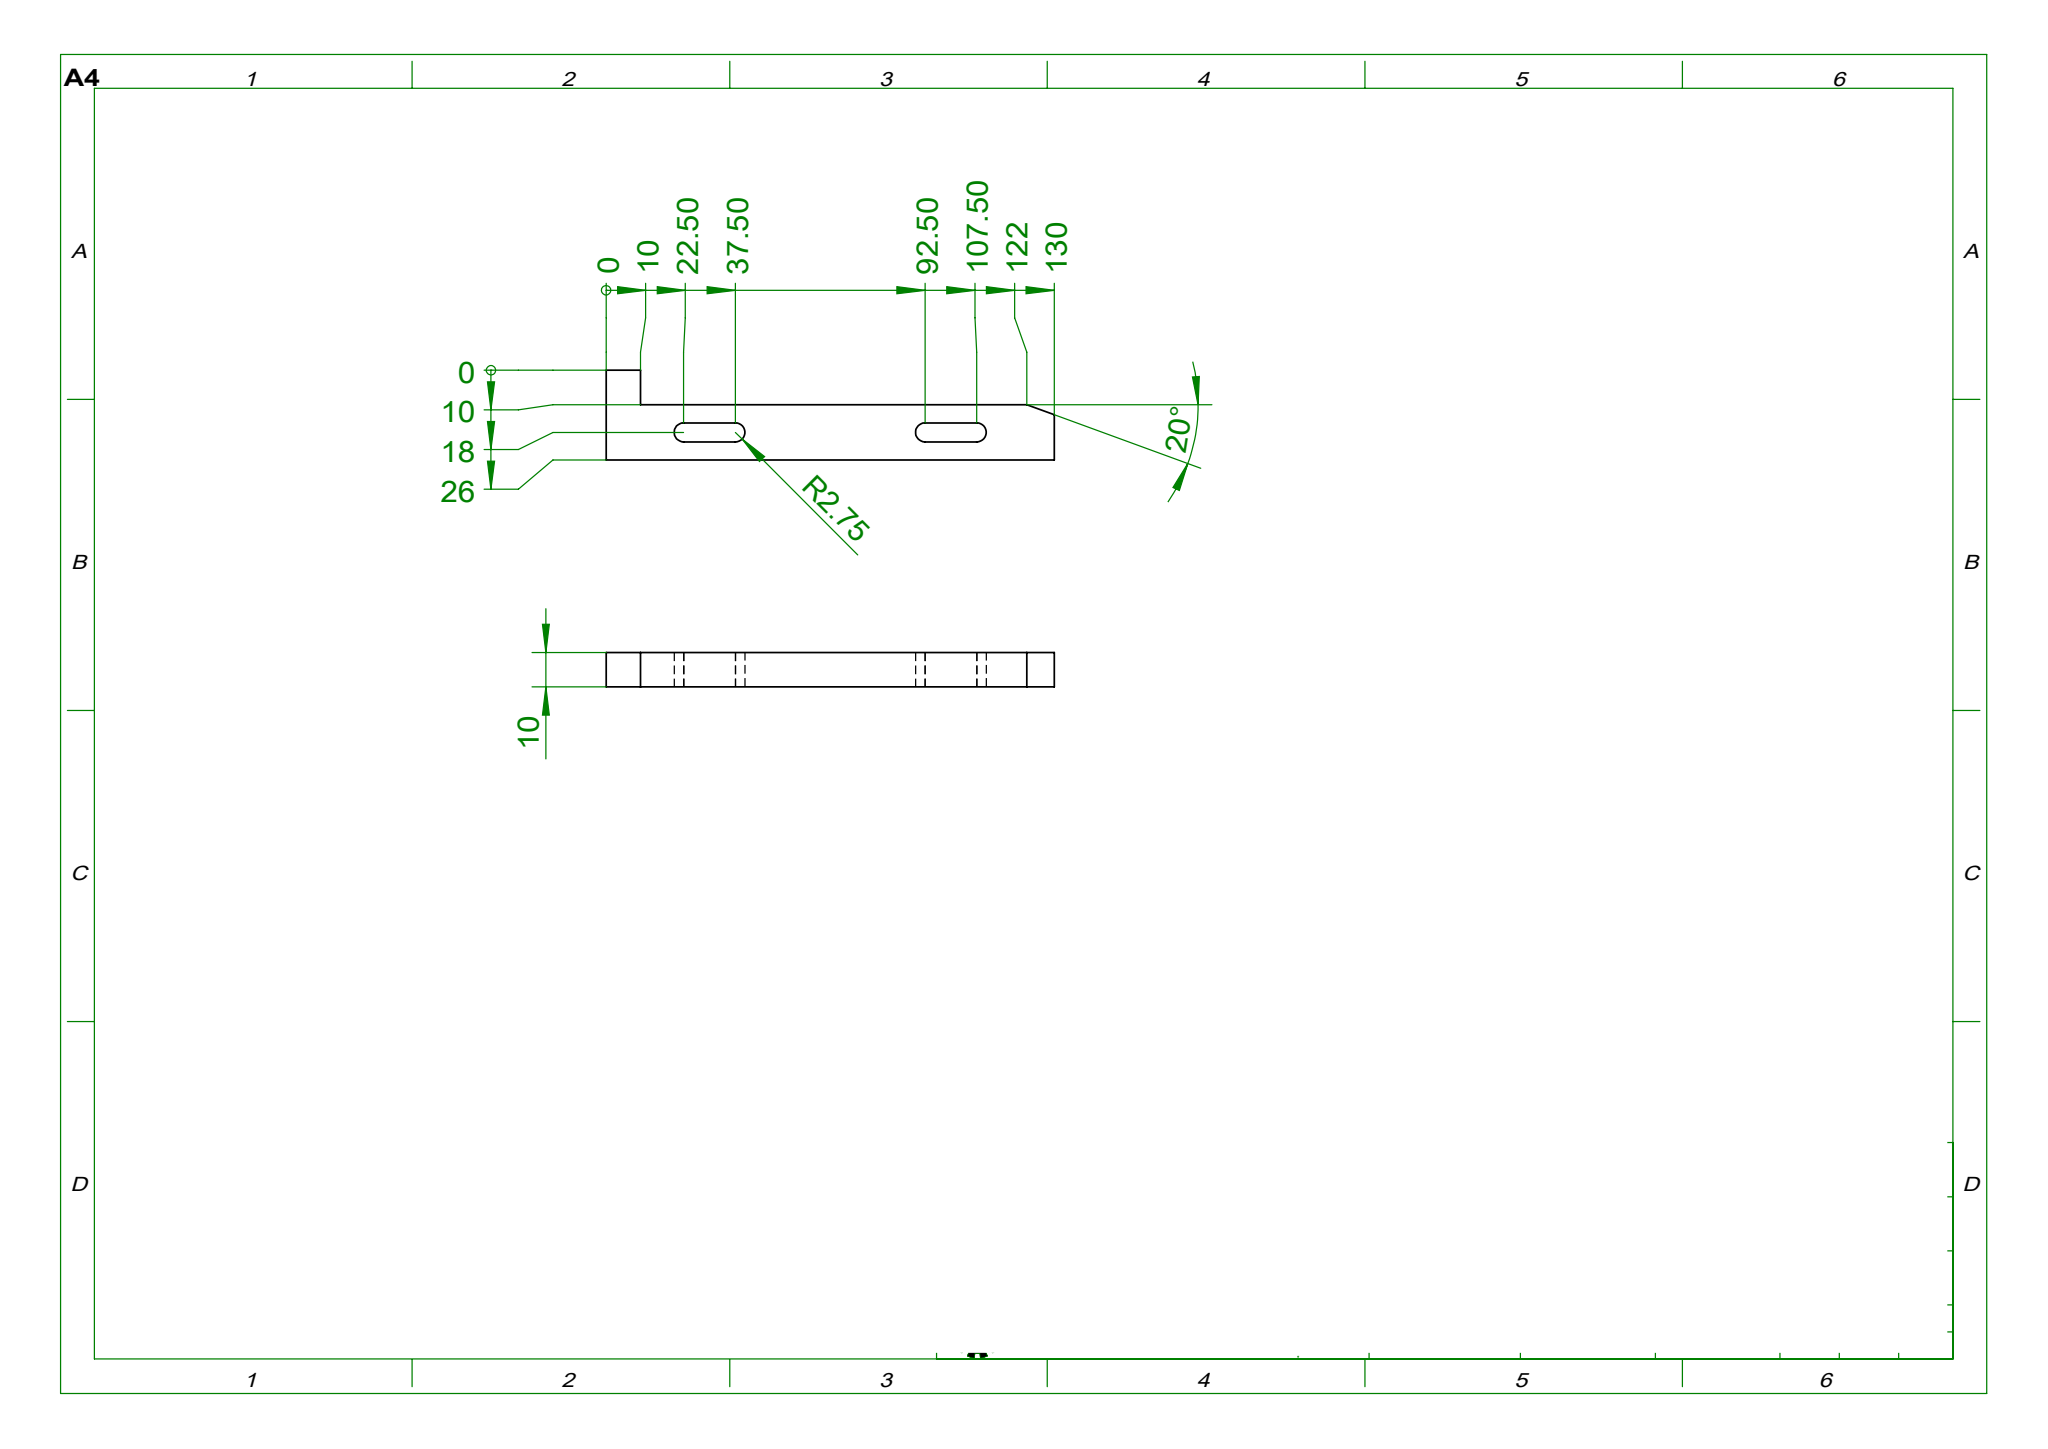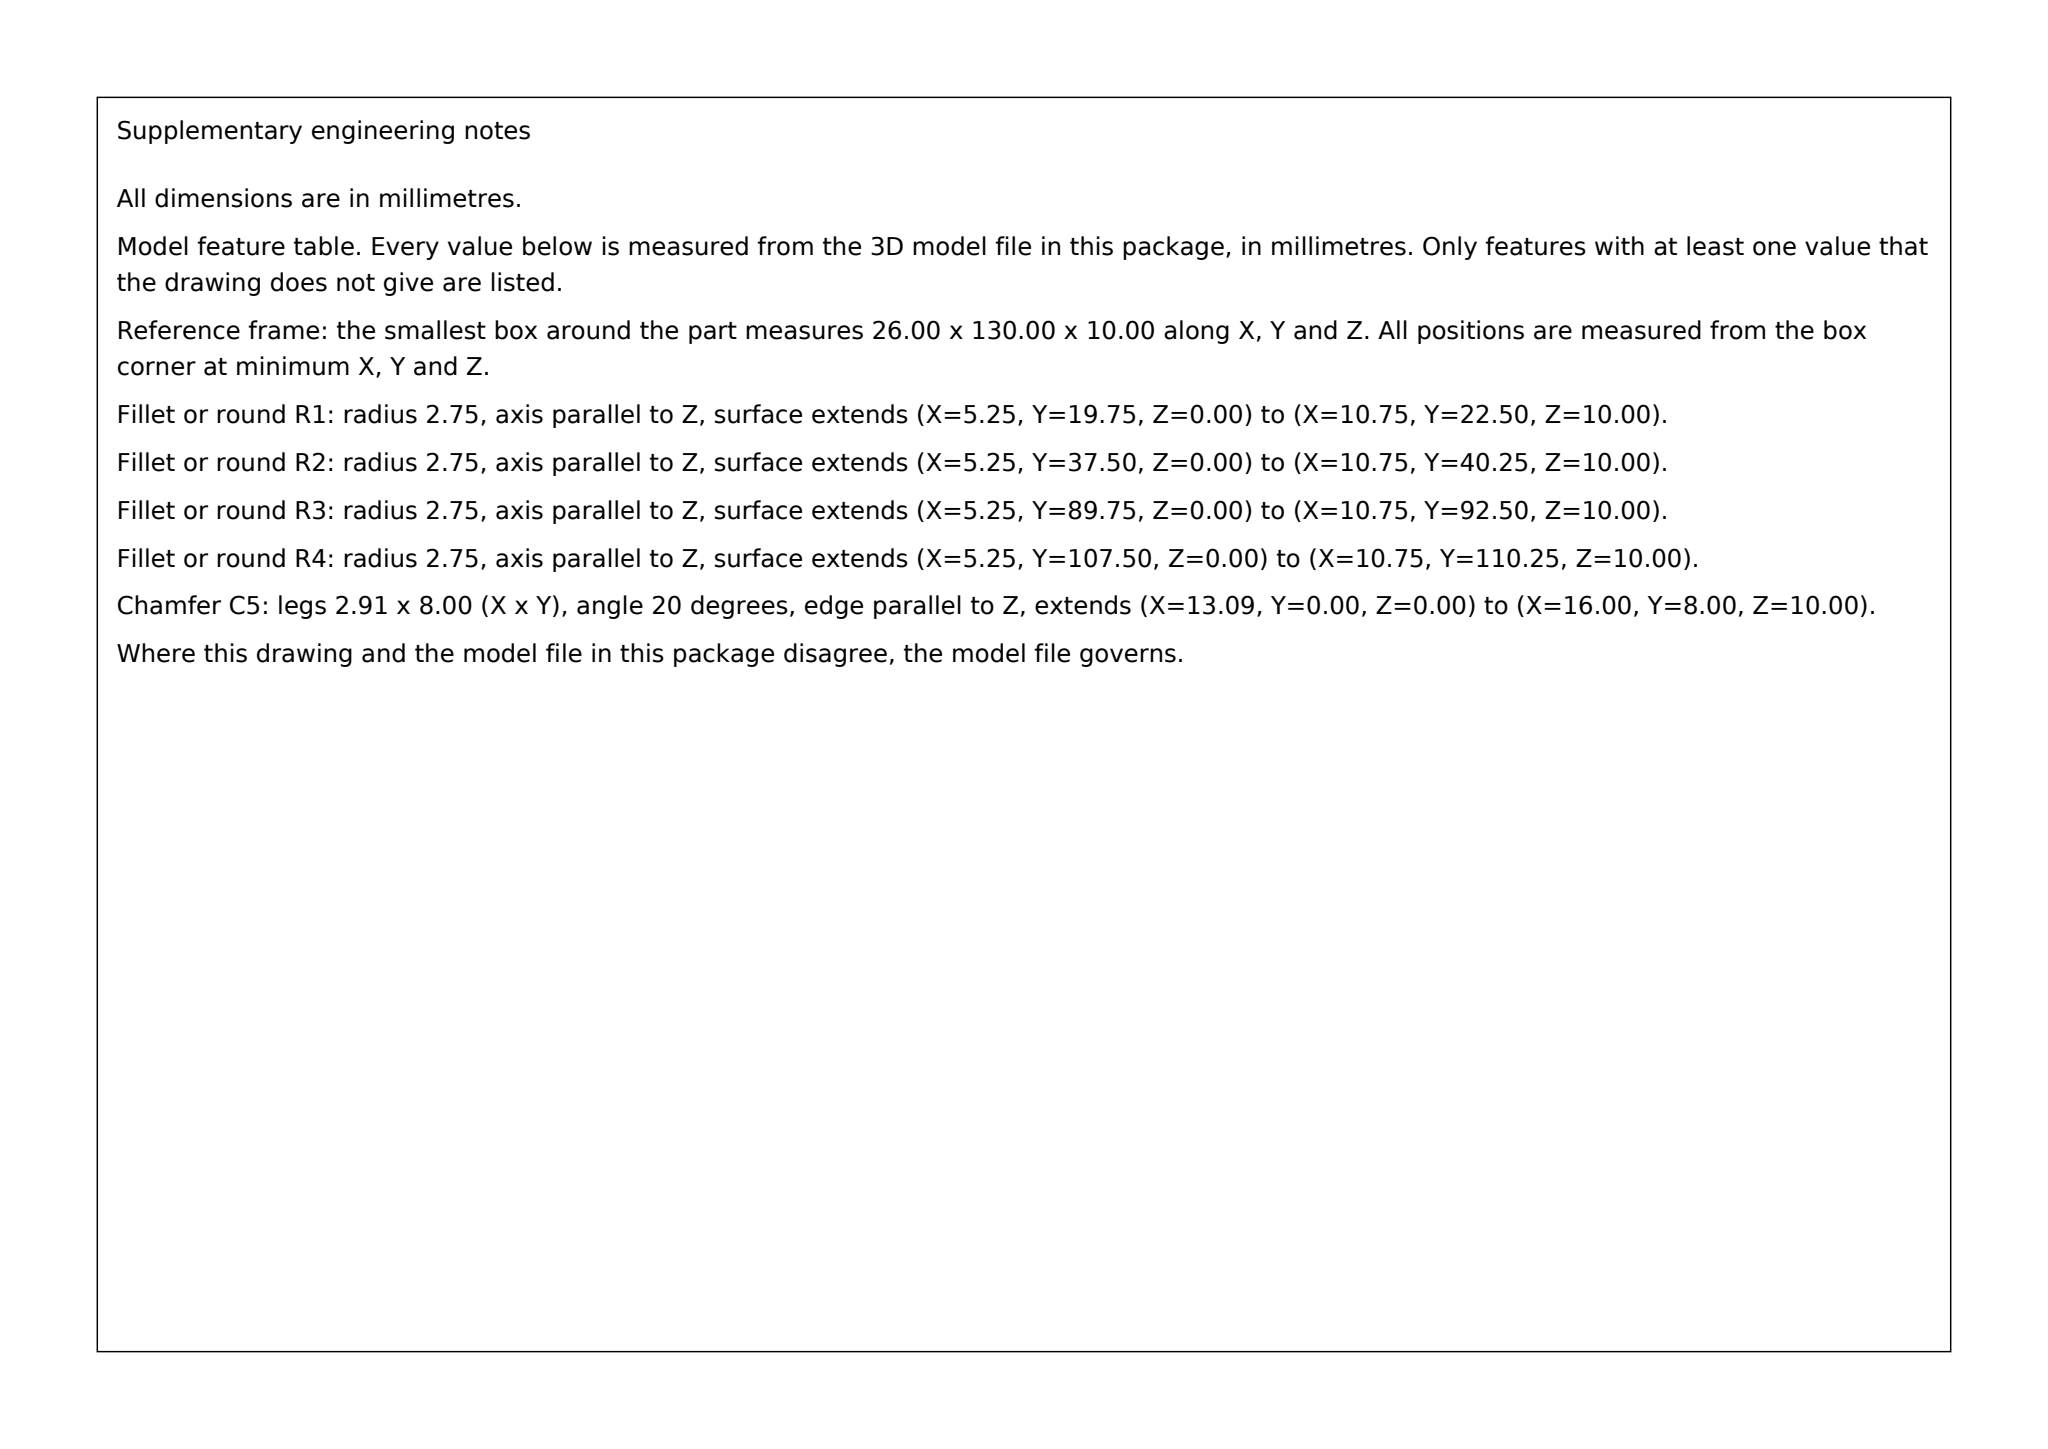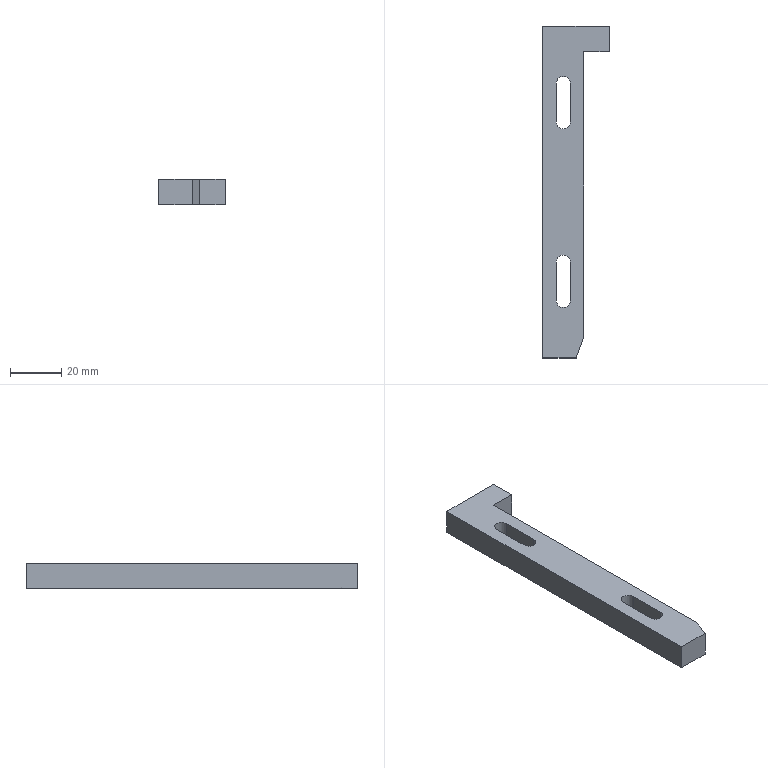Part | SolidWorks | mm | 1 solid | 17 faces | box 26 x 130 x 10 mm | volume 19558 mm3 | plane 13 | cylinder 4 | commonest cylinder face diameters 5.5 x4
build123d program:
from build123d import *

# Parameters (mm, degrees)
BOSS_EXTRUDE1_DEPTH = 10
CUT_EXTRUDE1_DEPTH  = 10
CHAMFER1_SIZE       = 8
CHAMFER1_SIZE2      = 2.912


with BuildPart() as part:
    # Sketch1 → Boss-Extrude1 (new body)
    with BuildSketch(Plane.XY):
        Polygon((16, 0), (16, 120), (26, 120), (26, 130), (0, 130), (0, 0), align=None)
    extrude(amount=BOSS_EXTRUDE1_DEPTH)

    # Sketch2 → Cut-Extrude1 (cut)
    with BuildSketch(Plane.XY.offset(10)):
        with BuildLine():
            Line((5.25, 22.5), (5.25, 37.5))
            ThreePointArc((5.25, 37.5), (8, 40.25), (10.75, 37.5))
            Line((10.75, 37.5), (10.75, 22.5))
            ThreePointArc((10.75, 22.5), (8, 19.75), (5.25, 22.5))
        make_face()
        with BuildLine():
            Line((5.25, 107.5), (5.25, 92.5))
            ThreePointArc((5.25, 92.5), (8, 89.75), (10.75, 92.5))
            Line((10.75, 92.5), (10.75, 107.5))
            ThreePointArc((10.75, 107.5), (8, 110.25), (5.25, 107.5))
        make_face()
    extrude(amount=-CUT_EXTRUDE1_DEPTH, mode=Mode.SUBTRACT)

    # Chamfer1
    chamfer1_edges = [part.edges().sort_by_distance(p)[0] for p in [
        (16, 0, 5),
    ]]
    chamfer1_side = [part.faces().sort_by_distance(p)[0] for p in [
        (16, 60, 5),
    ]]
    chamfer(chamfer1_edges, length=CHAMFER1_SIZE, length2=CHAMFER1_SIZE2, reference=chamfer1_side[0])


solid = part.part
STEP:
#1=CARTESIAN_POINT('',(0.,130.,0.));
#2=VERTEX_POINT('',#1);
#3=CARTESIAN_POINT('',(0.,0.,0.));
#4=VERTEX_POINT('',#3);
#5=CARTESIAN_POINT('',(0.,0.,0.));
#6=DIRECTION('',(0.,-1.,0.));
#7=VECTOR('',#6,1000.);
#8=LINE('',#5,#7);
#9=EDGE_CURVE('',#2,#4,#8,.T.);
#10=ORIENTED_EDGE('',*,*,#9,.T.);
#11=CARTESIAN_POINT('',(0.,0.,10.));
#12=VERTEX_POINT('',#11);
#13=CARTESIAN_POINT('',(0.,0.,10.));
#14=DIRECTION('',(0.,0.,-1.));
#15=VECTOR('',#14,1000.);
#16=LINE('',#13,#15);
#17=EDGE_CURVE('',#12,#4,#16,.T.);
#18=ORIENTED_EDGE('',*,*,#17,.F.);
#19=CARTESIAN_POINT('',(0.,130.,10.));
#20=VERTEX_POINT('',#19);
#21=CARTESIAN_POINT('',(0.,0.,10.));
#22=DIRECTION('',(0.,-1.,0.));
#23=VECTOR('',#22,1000.);
#24=LINE('',#21,#23);
#25=EDGE_CURVE('',#20,#12,#24,.T.);
#26=ORIENTED_EDGE('',*,*,#25,.F.);
#27=CARTESIAN_POINT('',(0.,130.,10.));
#28=DIRECTION('',(0.,0.,-1.));
#29=VECTOR('',#28,1000.);
#30=LINE('',#27,#29);
#31=EDGE_CURVE('',#20,#2,#30,.T.);
#32=ORIENTED_EDGE('',*,*,#31,.T.);
#33=EDGE_LOOP('',(#10,#18,#26,#32));
#34=FACE_OUTER_BOUND('',#33,.T.);
#35=CARTESIAN_POINT('',(0.,0.,10.));
#36=DIRECTION('',(1.,0.,0.));
#37=DIRECTION('',(0.,0.,-1.));
#38=AXIS2_PLACEMENT_3D('',#35,#36,#37);
#39=PLANE('',#38);
#40=ADVANCED_FACE('',(#34),#39,.F.);
#41=CARTESIAN_POINT('',(13.088,0.,0.));
#42=VERTEX_POINT('',#41);
#43=CARTESIAN_POINT('',(0.,0.,0.));
#44=DIRECTION('',(1.,0.,0.));
#45=VECTOR('',#44,1000.);
#46=LINE('',#43,#45);
#47=EDGE_CURVE('',#4,#42,#46,.T.);
#48=ORIENTED_EDGE('',*,*,#47,.T.);
#49=CARTESIAN_POINT('',(13.088,-0.,10.));
#50=VERTEX_POINT('',#49);
#51=CARTESIAN_POINT('',(13.088,0.,10.));
#52=DIRECTION('',(0.,0.,1.));
#53=VECTOR('',#52,1000.);
#54=LINE('',#51,#53);
#55=EDGE_CURVE('',#42,#50,#54,.T.);
#56=ORIENTED_EDGE('',*,*,#55,.T.);
#57=CARTESIAN_POINT('',(0.,0.,10.));
#58=DIRECTION('',(1.,0.,0.));
#59=VECTOR('',#58,1000.);
#60=LINE('',#57,#59);
#61=EDGE_CURVE('',#12,#50,#60,.T.);
#62=ORIENTED_EDGE('',*,*,#61,.F.);
#63=ORIENTED_EDGE('',*,*,#17,.T.);
#64=EDGE_LOOP('',(#48,#56,#62,#63));
#65=FACE_OUTER_BOUND('',#64,.T.);
#66=CARTESIAN_POINT('',(0.,0.,10.));
#67=DIRECTION('',(0.,1.,0.));
#68=DIRECTION('',(0.,0.,1.));
#69=AXIS2_PLACEMENT_3D('',#66,#67,#68);
#70=PLANE('',#69);
#71=ADVANCED_FACE('',(#65),#70,.F.);
#72=CARTESIAN_POINT('',(16.,8.,10.));
#73=VERTEX_POINT('',#72);
#74=CARTESIAN_POINT('',(16.,120.,10.));
#75=VERTEX_POINT('',#74);
#76=CARTESIAN_POINT('',(16.,0.,10.));
#77=DIRECTION('',(0.,1.,0.));
#78=VECTOR('',#77,1000.);
#79=LINE('',#76,#78);
#80=EDGE_CURVE('',#73,#75,#79,.T.);
#81=ORIENTED_EDGE('',*,*,#80,.F.);
#82=CARTESIAN_POINT('',(16.,8.,0.));
#83=VERTEX_POINT('',#82);
#84=CARTESIAN_POINT('',(16.,8.,10.));
#85=DIRECTION('',(0.,0.,-1.));
#86=VECTOR('',#85,1000.);
#87=LINE('',#84,#86);
#88=EDGE_CURVE('',#73,#83,#87,.T.);
#89=ORIENTED_EDGE('',*,*,#88,.T.);
#90=CARTESIAN_POINT('',(16.,120.,0.));
#91=VERTEX_POINT('',#90);
#92=CARTESIAN_POINT('',(16.,0.,0.));
#93=DIRECTION('',(0.,1.,0.));
#94=VECTOR('',#93,1000.);
#95=LINE('',#92,#94);
#96=EDGE_CURVE('',#83,#91,#95,.T.);
#97=ORIENTED_EDGE('',*,*,#96,.T.);
#98=CARTESIAN_POINT('',(16.,120.,10.));
#99=DIRECTION('',(0.,0.,-1.));
#100=VECTOR('',#99,1000.);
#101=LINE('',#98,#100);
#102=EDGE_CURVE('',#75,#91,#101,.T.);
#103=ORIENTED_EDGE('',*,*,#102,.F.);
#104=EDGE_LOOP('',(#81,#89,#97,#103));
#105=FACE_OUTER_BOUND('',#104,.T.);
#106=CARTESIAN_POINT('',(16.,0.,10.));
#107=DIRECTION('',(-1.,0.,0.));
#108=DIRECTION('',(0.,0.,1.));
#109=AXIS2_PLACEMENT_3D('',#106,#107,#108);
#110=PLANE('',#109);
#111=ADVANCED_FACE('',(#105),#110,.F.);
#112=CARTESIAN_POINT('',(26.,120.,0.));
#113=VERTEX_POINT('',#112);
#114=CARTESIAN_POINT('',(16.,120.,0.));
#115=DIRECTION('',(1.,0.,0.));
#116=VECTOR('',#115,1000.);
#117=LINE('',#114,#116);
#118=EDGE_CURVE('',#91,#113,#117,.T.);
#119=ORIENTED_EDGE('',*,*,#118,.T.);
#120=CARTESIAN_POINT('',(26.,120.,10.));
#121=VERTEX_POINT('',#120);
#122=CARTESIAN_POINT('',(26.,120.,10.));
#123=DIRECTION('',(0.,0.,-1.));
#124=VECTOR('',#123,1000.);
#125=LINE('',#122,#124);
#126=EDGE_CURVE('',#121,#113,#125,.T.);
#127=ORIENTED_EDGE('',*,*,#126,.F.);
#128=CARTESIAN_POINT('',(16.,120.,10.));
#129=DIRECTION('',(1.,0.,0.));
#130=VECTOR('',#129,1000.);
#131=LINE('',#128,#130);
#132=EDGE_CURVE('',#75,#121,#131,.T.);
#133=ORIENTED_EDGE('',*,*,#132,.F.);
#134=ORIENTED_EDGE('',*,*,#102,.T.);
#135=EDGE_LOOP('',(#119,#127,#133,#134));
#136=FACE_OUTER_BOUND('',#135,.T.);
#137=CARTESIAN_POINT('',(16.,120.,10.));
#138=DIRECTION('',(0.,1.,0.));
#139=DIRECTION('',(0.,0.,1.));
#140=AXIS2_PLACEMENT_3D('',#137,#138,#139);
#141=PLANE('',#140);
#142=ADVANCED_FACE('',(#136),#141,.F.);
#143=CARTESIAN_POINT('',(26.,130.,0.));
#144=VERTEX_POINT('',#143);
#145=CARTESIAN_POINT('',(26.,120.,0.));
#146=DIRECTION('',(0.,1.,0.));
#147=VECTOR('',#146,1000.);
#148=LINE('',#145,#147);
#149=EDGE_CURVE('',#113,#144,#148,.T.);
#150=ORIENTED_EDGE('',*,*,#149,.T.);
#151=CARTESIAN_POINT('',(26.,130.,10.));
#152=VERTEX_POINT('',#151);
#153=CARTESIAN_POINT('',(26.,130.,10.));
#154=DIRECTION('',(0.,0.,-1.));
#155=VECTOR('',#154,1000.);
#156=LINE('',#153,#155);
#157=EDGE_CURVE('',#152,#144,#156,.T.);
#158=ORIENTED_EDGE('',*,*,#157,.F.);
#159=CARTESIAN_POINT('',(26.,120.,10.));
#160=DIRECTION('',(0.,1.,0.));
#161=VECTOR('',#160,1000.);
#162=LINE('',#159,#161);
#163=EDGE_CURVE('',#121,#152,#162,.T.);
#164=ORIENTED_EDGE('',*,*,#163,.F.);
#165=ORIENTED_EDGE('',*,*,#126,.T.);
#166=EDGE_LOOP('',(#150,#158,#164,#165));
#167=FACE_OUTER_BOUND('',#166,.T.);
#168=CARTESIAN_POINT('',(26.,120.,10.));
#169=DIRECTION('',(-1.,0.,0.));
#170=DIRECTION('',(0.,0.,1.));
#171=AXIS2_PLACEMENT_3D('',#168,#169,#170);
#172=PLANE('',#171);
#173=ADVANCED_FACE('',(#167),#172,.F.);
#174=CARTESIAN_POINT('',(0.,130.,0.));
#175=DIRECTION('',(-1.,0.,0.));
#176=VECTOR('',#175,1000.);
#177=LINE('',#174,#176);
#178=EDGE_CURVE('',#144,#2,#177,.T.);
#179=ORIENTED_EDGE('',*,*,#178,.T.);
#180=ORIENTED_EDGE('',*,*,#31,.F.);
#181=CARTESIAN_POINT('',(0.,130.,10.));
#182=DIRECTION('',(-1.,0.,0.));
#183=VECTOR('',#182,1000.);
#184=LINE('',#181,#183);
#185=EDGE_CURVE('',#152,#20,#184,.T.);
#186=ORIENTED_EDGE('',*,*,#185,.F.);
#187=ORIENTED_EDGE('',*,*,#157,.T.);
#188=EDGE_LOOP('',(#179,#180,#186,#187));
#189=FACE_OUTER_BOUND('',#188,.T.);
#190=CARTESIAN_POINT('',(0.,130.,10.));
#191=DIRECTION('',(0.,-1.,0.));
#192=DIRECTION('',(0.,0.,-1.));
#193=AXIS2_PLACEMENT_3D('',#190,#191,#192);
#194=PLANE('',#193);
#195=ADVANCED_FACE('',(#189),#194,.F.);
#196=CARTESIAN_POINT('',(5.25,107.5,10.));
#197=VERTEX_POINT('',#196);
#198=CARTESIAN_POINT('',(5.25,92.5,10.));
#199=VERTEX_POINT('',#198);
#200=CARTESIAN_POINT('',(5.25,107.5,10.));
#201=DIRECTION('',(0.,-1.,0.));
#202=VECTOR('',#201,1000.);
#203=LINE('',#200,#202);
#204=EDGE_CURVE('',#197,#199,#203,.T.);
#205=ORIENTED_EDGE('',*,*,#204,.F.);
#206=CARTESIAN_POINT('',(10.75,107.5,10.));
#207=VERTEX_POINT('',#206);
#208=CARTESIAN_POINT('',(8.,107.5,10.));
#209=DIRECTION('',(0.,0.,1.));
#210=DIRECTION('',(-1.,0.,0.));
#211=AXIS2_PLACEMENT_3D('',#208,#209,#210);
#212=CIRCLE('',#211,2.75);
#213=EDGE_CURVE('',#207,#197,#212,.T.);
#214=ORIENTED_EDGE('',*,*,#213,.F.);
#215=CARTESIAN_POINT('',(10.75,92.5,10.));
#216=VERTEX_POINT('',#215);
#217=CARTESIAN_POINT('',(10.75,107.5,10.));
#218=DIRECTION('',(-0.,1.,0.));
#219=VECTOR('',#218,1000.);
#220=LINE('',#217,#219);
#221=EDGE_CURVE('',#216,#207,#220,.T.);
#222=ORIENTED_EDGE('',*,*,#221,.F.);
#223=CARTESIAN_POINT('',(8.,92.5,10.));
#224=DIRECTION('',(0.,0.,1.));
#225=DIRECTION('',(-1.,0.,0.));
#226=AXIS2_PLACEMENT_3D('',#223,#224,#225);
#227=CIRCLE('',#226,2.75);
#228=EDGE_CURVE('',#199,#216,#227,.T.);
#229=ORIENTED_EDGE('',*,*,#228,.F.);
#230=EDGE_LOOP('',(#205,#214,#222,#229));
#231=FACE_BOUND('',#230,.T.);
#232=CARTESIAN_POINT('',(10.75,22.5,10.));
#233=VERTEX_POINT('',#232);
#234=CARTESIAN_POINT('',(10.75,37.5,10.));
#235=VERTEX_POINT('',#234);
#236=CARTESIAN_POINT('',(10.75,22.5,10.));
#237=DIRECTION('',(0.,1.,0.));
#238=VECTOR('',#237,1000.);
#239=LINE('',#236,#238);
#240=EDGE_CURVE('',#233,#235,#239,.T.);
#241=ORIENTED_EDGE('',*,*,#240,.F.);
#242=CARTESIAN_POINT('',(5.25,22.5,10.));
#243=VERTEX_POINT('',#242);
#244=CARTESIAN_POINT('',(8.,22.5,10.));
#245=DIRECTION('',(0.,0.,1.));
#246=DIRECTION('',(1.,0.,0.));
#247=AXIS2_PLACEMENT_3D('',#244,#245,#246);
#248=CIRCLE('',#247,2.75);
#249=EDGE_CURVE('',#243,#233,#248,.T.);
#250=ORIENTED_EDGE('',*,*,#249,.F.);
#251=CARTESIAN_POINT('',(5.25,37.5,10.));
#252=VERTEX_POINT('',#251);
#253=CARTESIAN_POINT('',(5.25,22.5,10.));
#254=DIRECTION('',(-0.,-1.,0.));
#255=VECTOR('',#254,1000.);
#256=LINE('',#253,#255);
#257=EDGE_CURVE('',#252,#243,#256,.T.);
#258=ORIENTED_EDGE('',*,*,#257,.F.);
#259=CARTESIAN_POINT('',(8.,37.5,10.));
#260=DIRECTION('',(0.,0.,1.));
#261=DIRECTION('',(1.,0.,0.));
#262=AXIS2_PLACEMENT_3D('',#259,#260,#261);
#263=CIRCLE('',#262,2.75);
#264=EDGE_CURVE('',#235,#252,#263,.T.);
#265=ORIENTED_EDGE('',*,*,#264,.F.);
#266=EDGE_LOOP('',(#241,#250,#258,#265));
#267=FACE_BOUND('',#266,.T.);
#268=ORIENTED_EDGE('',*,*,#61,.T.);
#269=CARTESIAN_POINT('',(16.,8.,10.));
#270=DIRECTION('',(0.342,0.9397,0.));
#271=VECTOR('',#270,1000.);
#272=LINE('',#269,#271);
#273=EDGE_CURVE('',#50,#73,#272,.T.);
#274=ORIENTED_EDGE('',*,*,#273,.T.);
#275=ORIENTED_EDGE('',*,*,#80,.T.);
#276=ORIENTED_EDGE('',*,*,#132,.T.);
#277=ORIENTED_EDGE('',*,*,#163,.T.);
#278=ORIENTED_EDGE('',*,*,#185,.T.);
#279=ORIENTED_EDGE('',*,*,#25,.T.);
#280=EDGE_LOOP('',(#268,#274,#275,#276,#277,#278,#279));
#281=FACE_OUTER_BOUND('',#280,.T.);
#282=CARTESIAN_POINT('',(0.,0.,10.));
#283=DIRECTION('',(0.,0.,-1.));
#284=DIRECTION('',(-1.,0.,0.));
#285=AXIS2_PLACEMENT_3D('',#282,#283,#284);
#286=PLANE('',#285);
#287=ADVANCED_FACE('',(#231,#267,#281),#286,.F.);
#288=CARTESIAN_POINT('',(10.75,107.5,0.));
#289=VERTEX_POINT('',#288);
#290=CARTESIAN_POINT('',(5.25,107.5,0.));
#291=VERTEX_POINT('',#290);
#292=CARTESIAN_POINT('',(8.,107.5,0.));
#293=DIRECTION('',(0.,0.,1.));
#294=DIRECTION('',(-1.,0.,0.));
#295=AXIS2_PLACEMENT_3D('',#292,#293,#294);
#296=CIRCLE('',#295,2.75);
#297=EDGE_CURVE('',#289,#291,#296,.T.);
#298=ORIENTED_EDGE('',*,*,#297,.T.);
#299=CARTESIAN_POINT('',(5.25,92.5,0.));
#300=VERTEX_POINT('',#299);
#301=CARTESIAN_POINT('',(5.25,107.5,0.));
#302=DIRECTION('',(0.,-1.,0.));
#303=VECTOR('',#302,1000.);
#304=LINE('',#301,#303);
#305=EDGE_CURVE('',#291,#300,#304,.T.);
#306=ORIENTED_EDGE('',*,*,#305,.T.);
#307=CARTESIAN_POINT('',(10.75,92.5,0.));
#308=VERTEX_POINT('',#307);
#309=CARTESIAN_POINT('',(8.,92.5,0.));
#310=DIRECTION('',(0.,0.,1.));
#311=DIRECTION('',(-1.,0.,0.));
#312=AXIS2_PLACEMENT_3D('',#309,#310,#311);
#313=CIRCLE('',#312,2.75);
#314=EDGE_CURVE('',#300,#308,#313,.T.);
#315=ORIENTED_EDGE('',*,*,#314,.T.);
#316=CARTESIAN_POINT('',(10.75,107.5,0.));
#317=DIRECTION('',(-0.,1.,0.));
#318=VECTOR('',#317,1000.);
#319=LINE('',#316,#318);
#320=EDGE_CURVE('',#308,#289,#319,.T.);
#321=ORIENTED_EDGE('',*,*,#320,.T.);
#322=EDGE_LOOP('',(#298,#306,#315,#321));
#323=FACE_BOUND('',#322,.T.);
#324=CARTESIAN_POINT('',(5.25,22.5,0.));
#325=VERTEX_POINT('',#324);
#326=CARTESIAN_POINT('',(10.75,22.5,0.));
#327=VERTEX_POINT('',#326);
#328=CARTESIAN_POINT('',(8.,22.5,0.));
#329=DIRECTION('',(0.,0.,1.));
#330=DIRECTION('',(1.,0.,0.));
#331=AXIS2_PLACEMENT_3D('',#328,#329,#330);
#332=CIRCLE('',#331,2.75);
#333=EDGE_CURVE('',#325,#327,#332,.T.);
#334=ORIENTED_EDGE('',*,*,#333,.T.);
#335=CARTESIAN_POINT('',(10.75,37.5,0.));
#336=VERTEX_POINT('',#335);
#337=CARTESIAN_POINT('',(10.75,22.5,0.));
#338=DIRECTION('',(0.,1.,0.));
#339=VECTOR('',#338,1000.);
#340=LINE('',#337,#339);
#341=EDGE_CURVE('',#327,#336,#340,.T.);
#342=ORIENTED_EDGE('',*,*,#341,.T.);
#343=CARTESIAN_POINT('',(5.25,37.5,0.));
#344=VERTEX_POINT('',#343);
#345=CARTESIAN_POINT('',(8.,37.5,0.));
#346=DIRECTION('',(0.,0.,1.));
#347=DIRECTION('',(1.,0.,0.));
#348=AXIS2_PLACEMENT_3D('',#345,#346,#347);
#349=CIRCLE('',#348,2.75);
#350=EDGE_CURVE('',#336,#344,#349,.T.);
#351=ORIENTED_EDGE('',*,*,#350,.T.);
#352=CARTESIAN_POINT('',(5.25,22.5,0.));
#353=DIRECTION('',(-0.,-1.,0.));
#354=VECTOR('',#353,1000.);
#355=LINE('',#352,#354);
#356=EDGE_CURVE('',#344,#325,#355,.T.);
#357=ORIENTED_EDGE('',*,*,#356,.T.);
#358=EDGE_LOOP('',(#334,#342,#351,#357));
#359=FACE_BOUND('',#358,.T.);
#360=ORIENTED_EDGE('',*,*,#96,.F.);
#361=CARTESIAN_POINT('',(11.557,-4.206,0.));
#362=DIRECTION('',(-0.342,-0.9397,0.));
#363=VECTOR('',#362,1000.);
#364=LINE('',#361,#363);
#365=EDGE_CURVE('',#83,#42,#364,.T.);
#366=ORIENTED_EDGE('',*,*,#365,.T.);
#367=ORIENTED_EDGE('',*,*,#47,.F.);
#368=ORIENTED_EDGE('',*,*,#9,.F.);
#369=ORIENTED_EDGE('',*,*,#178,.F.);
#370=ORIENTED_EDGE('',*,*,#149,.F.);
#371=ORIENTED_EDGE('',*,*,#118,.F.);
#372=EDGE_LOOP('',(#360,#366,#367,#368,#369,#370,#371));
#373=FACE_OUTER_BOUND('',#372,.T.);
#374=CARTESIAN_POINT('',(0.,0.,0.));
#375=DIRECTION('',(0.,0.,-1.));
#376=DIRECTION('',(-1.,0.,0.));
#377=AXIS2_PLACEMENT_3D('',#374,#375,#376);
#378=PLANE('',#377);
#379=ADVANCED_FACE('',(#323,#359,#373),#378,.T.);
#380=ORIENTED_EDGE('',*,*,#249,.T.);
#381=CARTESIAN_POINT('',(10.75,22.5,0.));
#382=DIRECTION('',(0.,0.,1.));
#383=VECTOR('',#382,1000.);
#384=LINE('',#381,#383);
#385=EDGE_CURVE('',#327,#233,#384,.T.);
#386=ORIENTED_EDGE('',*,*,#385,.F.);
#387=ORIENTED_EDGE('',*,*,#333,.F.);
#388=CARTESIAN_POINT('',(5.25,22.5,0.));
#389=DIRECTION('',(0.,0.,1.));
#390=VECTOR('',#389,1000.);
#391=LINE('',#388,#390);
#392=EDGE_CURVE('',#325,#243,#391,.T.);
#393=ORIENTED_EDGE('',*,*,#392,.T.);
#394=EDGE_LOOP('',(#380,#386,#387,#393));
#395=FACE_OUTER_BOUND('',#394,.T.);
#396=CARTESIAN_POINT('',(8.,22.5,0.));
#397=DIRECTION('',(0.,0.,1.));
#398=DIRECTION('',(1.,0.,0.));
#399=AXIS2_PLACEMENT_3D('',#396,#397,#398);
#400=CYLINDRICAL_SURFACE('',#399,2.75);
#401=ADVANCED_FACE('',(#395),#400,.F.);
#402=ORIENTED_EDGE('',*,*,#257,.T.);
#403=ORIENTED_EDGE('',*,*,#392,.F.);
#404=ORIENTED_EDGE('',*,*,#356,.F.);
#405=CARTESIAN_POINT('',(5.25,37.5,0.));
#406=DIRECTION('',(0.,0.,1.));
#407=VECTOR('',#406,1000.);
#408=LINE('',#405,#407);
#409=EDGE_CURVE('',#344,#252,#408,.T.);
#410=ORIENTED_EDGE('',*,*,#409,.T.);
#411=EDGE_LOOP('',(#402,#403,#404,#410));
#412=FACE_OUTER_BOUND('',#411,.T.);
#413=CARTESIAN_POINT('',(5.25,22.5,0.));
#414=DIRECTION('',(-1.,0.,0.));
#415=DIRECTION('',(-0.,-1.,0.));
#416=AXIS2_PLACEMENT_3D('',#413,#414,#415);
#417=PLANE('',#416);
#418=ADVANCED_FACE('',(#412),#417,.F.);
#419=ORIENTED_EDGE('',*,*,#264,.T.);
#420=ORIENTED_EDGE('',*,*,#409,.F.);
#421=ORIENTED_EDGE('',*,*,#350,.F.);
#422=CARTESIAN_POINT('',(10.75,37.5,0.));
#423=DIRECTION('',(0.,0.,1.));
#424=VECTOR('',#423,1000.);
#425=LINE('',#422,#424);
#426=EDGE_CURVE('',#336,#235,#425,.T.);
#427=ORIENTED_EDGE('',*,*,#426,.T.);
#428=EDGE_LOOP('',(#419,#420,#421,#427));
#429=FACE_OUTER_BOUND('',#428,.T.);
#430=CARTESIAN_POINT('',(8.,37.5,0.));
#431=DIRECTION('',(0.,0.,1.));
#432=DIRECTION('',(1.,0.,0.));
#433=AXIS2_PLACEMENT_3D('',#430,#431,#432);
#434=CYLINDRICAL_SURFACE('',#433,2.75);
#435=ADVANCED_FACE('',(#429),#434,.F.);
#436=ORIENTED_EDGE('',*,*,#240,.T.);
#437=ORIENTED_EDGE('',*,*,#426,.F.);
#438=ORIENTED_EDGE('',*,*,#341,.F.);
#439=ORIENTED_EDGE('',*,*,#385,.T.);
#440=EDGE_LOOP('',(#436,#437,#438,#439));
#441=FACE_OUTER_BOUND('',#440,.T.);
#442=CARTESIAN_POINT('',(10.75,22.5,0.));
#443=DIRECTION('',(1.,-0.,0.));
#444=DIRECTION('',(0.,1.,0.));
#445=AXIS2_PLACEMENT_3D('',#442,#443,#444);
#446=PLANE('',#445);
#447=ADVANCED_FACE('',(#441),#446,.F.);
#448=ORIENTED_EDGE('',*,*,#213,.T.);
#449=CARTESIAN_POINT('',(5.25,107.5,0.));
#450=DIRECTION('',(0.,0.,1.));
#451=VECTOR('',#450,1000.);
#452=LINE('',#449,#451);
#453=EDGE_CURVE('',#291,#197,#452,.T.);
#454=ORIENTED_EDGE('',*,*,#453,.F.);
#455=ORIENTED_EDGE('',*,*,#297,.F.);
#456=CARTESIAN_POINT('',(10.75,107.5,0.));
#457=DIRECTION('',(0.,0.,1.));
#458=VECTOR('',#457,1000.);
#459=LINE('',#456,#458);
#460=EDGE_CURVE('',#289,#207,#459,.T.);
#461=ORIENTED_EDGE('',*,*,#460,.T.);
#462=EDGE_LOOP('',(#448,#454,#455,#461));
#463=FACE_OUTER_BOUND('',#462,.T.);
#464=CARTESIAN_POINT('',(8.,107.5,0.));
#465=DIRECTION('',(0.,0.,1.));
#466=DIRECTION('',(1.,0.,0.));
#467=AXIS2_PLACEMENT_3D('',#464,#465,#466);
#468=CYLINDRICAL_SURFACE('',#467,2.75);
#469=ADVANCED_FACE('',(#463),#468,.F.);
#470=ORIENTED_EDGE('',*,*,#221,.T.);
#471=ORIENTED_EDGE('',*,*,#460,.F.);
#472=ORIENTED_EDGE('',*,*,#320,.F.);
#473=CARTESIAN_POINT('',(10.75,92.5,0.));
#474=DIRECTION('',(0.,0.,1.));
#475=VECTOR('',#474,1000.);
#476=LINE('',#473,#475);
#477=EDGE_CURVE('',#308,#216,#476,.T.);
#478=ORIENTED_EDGE('',*,*,#477,.T.);
#479=EDGE_LOOP('',(#470,#471,#472,#478));
#480=FACE_OUTER_BOUND('',#479,.T.);
#481=CARTESIAN_POINT('',(10.75,107.5,0.));
#482=DIRECTION('',(1.,0.,0.));
#483=DIRECTION('',(-0.,1.,0.));
#484=AXIS2_PLACEMENT_3D('',#481,#482,#483);
#485=PLANE('',#484);
#486=ADVANCED_FACE('',(#480),#485,.F.);
#487=ORIENTED_EDGE('',*,*,#228,.T.);
#488=ORIENTED_EDGE('',*,*,#477,.F.);
#489=ORIENTED_EDGE('',*,*,#314,.F.);
#490=CARTESIAN_POINT('',(5.25,92.5,0.));
#491=DIRECTION('',(0.,0.,1.));
#492=VECTOR('',#491,1000.);
#493=LINE('',#490,#492);
#494=EDGE_CURVE('',#300,#199,#493,.T.);
#495=ORIENTED_EDGE('',*,*,#494,.T.);
#496=EDGE_LOOP('',(#487,#488,#489,#495));
#497=FACE_OUTER_BOUND('',#496,.T.);
#498=CARTESIAN_POINT('',(8.,92.5,0.));
#499=DIRECTION('',(0.,0.,1.));
#500=DIRECTION('',(1.,0.,0.));
#501=AXIS2_PLACEMENT_3D('',#498,#499,#500);
#502=CYLINDRICAL_SURFACE('',#501,2.75);
#503=ADVANCED_FACE('',(#497),#502,.F.);
#504=ORIENTED_EDGE('',*,*,#204,.T.);
#505=ORIENTED_EDGE('',*,*,#494,.F.);
#506=ORIENTED_EDGE('',*,*,#305,.F.);
#507=ORIENTED_EDGE('',*,*,#453,.T.);
#508=EDGE_LOOP('',(#504,#505,#506,#507));
#509=FACE_OUTER_BOUND('',#508,.T.);
#510=CARTESIAN_POINT('',(5.25,107.5,0.));
#511=DIRECTION('',(-1.,-0.,0.));
#512=DIRECTION('',(0.,-1.,0.));
#513=AXIS2_PLACEMENT_3D('',#510,#511,#512);
#514=PLANE('',#513);
#515=ADVANCED_FACE('',(#509),#514,.F.);
#516=ORIENTED_EDGE('',*,*,#273,.F.);
#517=ORIENTED_EDGE('',*,*,#55,.F.);
#518=ORIENTED_EDGE('',*,*,#365,.F.);
#519=ORIENTED_EDGE('',*,*,#88,.F.);
#520=EDGE_LOOP('',(#516,#517,#518,#519));
#521=FACE_OUTER_BOUND('',#520,.T.);
#522=CARTESIAN_POINT('',(16.,8.,10.));
#523=DIRECTION('',(-0.9397,0.342,0.));
#524=DIRECTION('',(0.,0.,-1.));
#525=AXIS2_PLACEMENT_3D('',#522,#523,#524);
#526=PLANE('',#525);
#527=ADVANCED_FACE('',(#521),#526,.F.);
#528=CLOSED_SHELL('',(#40,#71,#111,#142,#173,#195,#287,#379,#401,#418,#435,#447,#469,#486,#503,#515,#527));
#529=MANIFOLD_SOLID_BREP('',#528);
#530=CARTESIAN_POINT('',(0.,0.,0.));
#531=DIRECTION('',(0.,0.,1.));
#532=DIRECTION('',(1.,0.,0.));
#533=AXIS2_PLACEMENT_3D('',#530,#531,#532);
#534=(LENGTH_UNIT()NAMED_UNIT(*)SI_UNIT(.MILLI.,.METRE.));
#535=UNCERTAINTY_MEASURE_WITH_UNIT(LENGTH_MEASURE(0.00001),#534,'','');
#536=(NAMED_UNIT(*)PLANE_ANGLE_UNIT()SI_UNIT($,.RADIAN.));
#537=(NAMED_UNIT(*)SI_UNIT($,.STERADIAN.)SOLID_ANGLE_UNIT());
#538=(GEOMETRIC_REPRESENTATION_CONTEXT(3)GLOBAL_UNCERTAINTY_ASSIGNED_CONTEXT((#535))GLOBAL_UNIT_ASSIGNED_CONTEXT((#534,#536,#537))REPRESENTATION_CONTEXT('',''));
#539=ADVANCED_BREP_SHAPE_REPRESENTATION('',(#529,#533),#538);